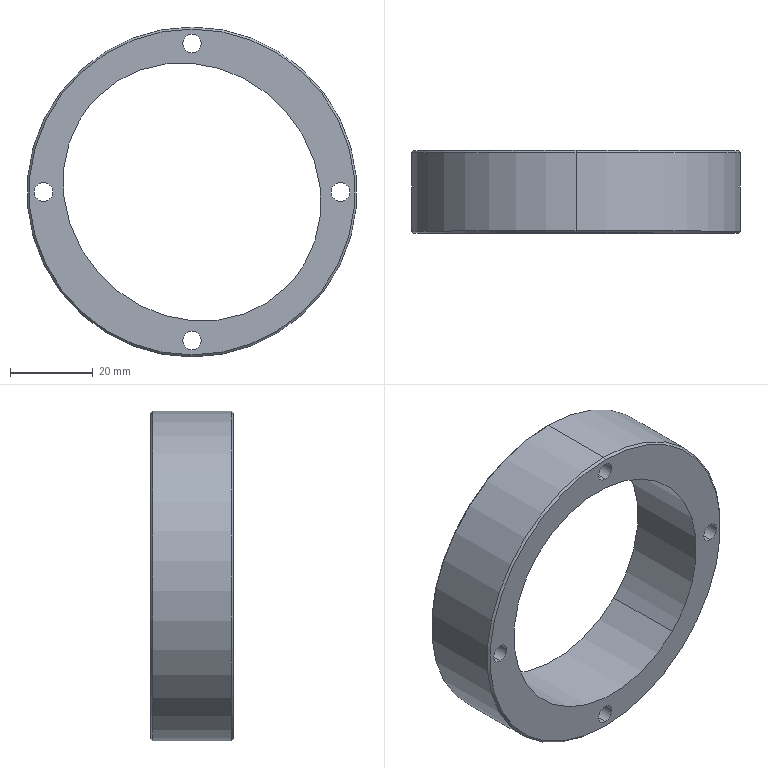Component | SolidWorks | 2-1 | 1 solid | 18 faces | box 80 x 20 x 80 mm | volume 37935 mm3 | cylinder 10 | cone 4 | spline 2 | plane 2 | commonest cylinder face diameters 4.5 x8 80 x2
build123d program:
from build123d import *

# Parameters (mm, degrees)
SKETCH1_R           = 40
BOSS_EXTRUDE1_DEPTH = 20
SKETCH2_R           = 2.25
CUT_EXTRUDE1_DEPTH  = 110
SKETCH3_RX          = 32.5
SKETCH3_RY          = 30
CUT_EXTRUDE2_DEPTH  = 110
CHAMFER1_SIZE       = 0.5


with BuildPart() as part:
    # Sketch1 → Boss-Extrude1 (new body)
    with BuildSketch(Plane(origin=(0, 0, 0), x_dir=(1, 0, 0), z_dir=(0, 1, 0))):
        with Locations(Location((0, 0, 0), (0, 0, 270))):
            Circle(SKETCH1_R)
    extrude(amount=BOSS_EXTRUDE1_DEPTH)

    # Sketch2 → Cut-Extrude1 (cut)
    with BuildSketch(Plane(origin=(0, 20, 0), x_dir=(1, 0, 0), z_dir=(0, 1, 0))):
        with Locations(Location((0, 36, 0), (0, 0, 270))):
            Circle(SKETCH2_R)
        with Locations(Location((36, 0, 0), (0, 0, 270))):
            Circle(SKETCH2_R)
        with Locations(Location((0, -36, 0), (0, 0, 270))):
            Circle(SKETCH2_R)
        with Locations(Location((-36, 0, 0), (0, 0, 270))):
            Circle(SKETCH2_R)
    extrude(amount=-CUT_EXTRUDE1_DEPTH, mode=Mode.SUBTRACT)

    # Sketch3 → Cut-Extrude2 (cut)
    with BuildSketch(Plane(origin=(0, 20, 0), x_dir=(1, 0, 0), z_dir=(0, 1, 0))):
        with Locations(Location((0, 0), (0, 0, 45))):
            Ellipse(SKETCH3_RX, SKETCH3_RY)
    extrude(amount=-CUT_EXTRUDE2_DEPTH, mode=Mode.SUBTRACT)

    # Chamfer1
    chamfer1_edges = [part.edges().sort_by_distance(p)[0] for p in [
        (0, 0, -40),
        (0, 20, -40),
    ]]
    chamfer(chamfer1_edges, length=CHAMFER1_SIZE)


solid = part.part

# Placed as in the assembly
solid = solid.moved(Location((0.004478, 20, 0), (0, 0, 0)))
STEP:
#1=COLOUR_RGB('',0.7922,0.8196,0.9333);
#2=FILL_AREA_STYLE_COLOUR('',#1);
#3=FILL_AREA_STYLE('',(#2));
#4=SURFACE_STYLE_FILL_AREA(#3);
#5=SURFACE_SIDE_STYLE('',(#4));
#6=SURFACE_STYLE_USAGE(.BOTH.,#5);
#7=PRESENTATION_STYLE_ASSIGNMENT((#6));
#8=CARTESIAN_POINT('',(0.,1.575,1.555));
#9=VERTEX_POINT('',#8);
#10=CARTESIAN_POINT('',(0.,1.575,-1.555));
#11=VERTEX_POINT('',#10);
#12=CARTESIAN_POINT('',(0.,1.575,0.));
#13=DIRECTION('',(0.,1.,0.));
#14=DIRECTION('',(0.,0.,1.));
#15=AXIS2_PLACEMENT_3D('',#12,#13,#14);
#16=CIRCLE('',#15,1.555);
#17=EDGE_CURVE('',#9,#11,#16,.T.);
#18=ORIENTED_EDGE('',*,*,#17,.F.);
#19=CARTESIAN_POINT('',(0.,1.555,1.575));
#20=VERTEX_POINT('',#19);
#21=CARTESIAN_POINT('',(0.,1.575,1.555));
#22=DIRECTION('',(0.,-0.7071,0.7071));
#23=VECTOR('',#22,39.37);
#24=LINE('',#21,#23);
#25=EDGE_CURVE('',#9,#20,#24,.T.);
#26=ORIENTED_EDGE('',*,*,#25,.T.);
#27=CARTESIAN_POINT('',(0.,1.555,-1.575));
#28=VERTEX_POINT('',#27);
#29=CARTESIAN_POINT('',(0.,1.555,0.));
#30=DIRECTION('',(0.,-1.,0.));
#31=DIRECTION('',(0.,0.,1.));
#32=AXIS2_PLACEMENT_3D('',#29,#30,#31);
#33=CIRCLE('',#32,1.575);
#34=EDGE_CURVE('',#28,#20,#33,.T.);
#35=ORIENTED_EDGE('',*,*,#34,.F.);
#36=CARTESIAN_POINT('',(0.,1.575,-1.555));
#37=DIRECTION('',(0.,-0.7071,-0.7071));
#38=VECTOR('',#37,39.37);
#39=LINE('',#36,#38);
#40=EDGE_CURVE('',#11,#28,#39,.T.);
#41=ORIENTED_EDGE('',*,*,#40,.F.);
#42=EDGE_LOOP('',(#18,#26,#35,#41));
#43=FACE_OUTER_BOUND('',#42,.T.);
#44=CARTESIAN_POINT('',(0.,1.575,0.));
#45=DIRECTION('',(0.,-1.,0.));
#46=DIRECTION('',(0.,0.,-1.));
#47=AXIS2_PLACEMENT_3D('',#44,#45,#46);
#48=CONICAL_SURFACE('',#47,1.555,0.7854);
#49=ADVANCED_FACE('',(#43),#48,.T.);
#50=CARTESIAN_POINT('',(0.,0.7874,-1.555));
#51=VERTEX_POINT('',#50);
#52=CARTESIAN_POINT('',(0.,0.7874,1.555));
#53=VERTEX_POINT('',#52);
#54=CARTESIAN_POINT('',(0.,0.7874,0.));
#55=DIRECTION('',(0.,-1.,0.));
#56=DIRECTION('',(0.,0.,1.));
#57=AXIS2_PLACEMENT_3D('',#54,#55,#56);
#58=CIRCLE('',#57,1.555);
#59=EDGE_CURVE('',#51,#53,#58,.T.);
#60=ORIENTED_EDGE('',*,*,#59,.F.);
#61=CARTESIAN_POINT('',(0.,0.8071,-1.575));
#62=VERTEX_POINT('',#61);
#63=CARTESIAN_POINT('',(0.,0.8071,-1.575));
#64=DIRECTION('',(0.,0.7071,-0.7071));
#65=VECTOR('',#64,39.37);
#66=LINE('',#63,#65);
#67=EDGE_CURVE('',#51,#62,#66,.T.);
#68=ORIENTED_EDGE('',*,*,#67,.T.);
#69=CARTESIAN_POINT('',(0.,0.8071,1.575));
#70=VERTEX_POINT('',#69);
#71=CARTESIAN_POINT('',(0.,0.8071,0.));
#72=DIRECTION('',(0.,1.,0.));
#73=DIRECTION('',(0.,0.,1.));
#74=AXIS2_PLACEMENT_3D('',#71,#72,#73);
#75=CIRCLE('',#74,1.575);
#76=EDGE_CURVE('',#70,#62,#75,.T.);
#77=ORIENTED_EDGE('',*,*,#76,.F.);
#78=CARTESIAN_POINT('',(0.,0.8071,1.575));
#79=DIRECTION('',(0.,0.7071,0.7071));
#80=VECTOR('',#79,39.37);
#81=LINE('',#78,#80);
#82=EDGE_CURVE('',#53,#70,#81,.T.);
#83=ORIENTED_EDGE('',*,*,#82,.F.);
#84=EDGE_LOOP('',(#60,#68,#77,#83));
#85=FACE_OUTER_BOUND('',#84,.T.);
#86=CARTESIAN_POINT('',(0.,0.8071,0.));
#87=DIRECTION('',(0.,1.,0.));
#88=DIRECTION('',(0.,0.,1.));
#89=AXIS2_PLACEMENT_3D('',#86,#87,#88);
#90=CONICAL_SURFACE('',#89,1.575,0.7854);
#91=ADVANCED_FACE('',(#85),#90,.T.);
#92=CARTESIAN_POINT('',(-0.9048,0.7874,0.9048));
#93=VERTEX_POINT('',#92);
#94=CARTESIAN_POINT('',(0.9048,0.7874,-0.9048));
#95=VERTEX_POINT('',#94);
#96=CARTESIAN_POINT('',(-0.9048,0.7874,0.9048));
#97=CARTESIAN_POINT('',(0.7656,0.7874,2.575));
#98=CARTESIAN_POINT('',(2.575,0.7874,0.7656));
#99=CARTESIAN_POINT('',(0.9048,0.7874,-0.9048));
#100=(BOUNDED_CURVE()B_SPLINE_CURVE(3,(#96,#97,#98,#99),.UNSPECIFIED.,.F.,.F.)B_SPLINE_CURVE_WITH_KNOTS((4,4),(3.142,6.283),.UNSPECIFIED.)CURVE()GEOMETRIC_REPRESENTATION_ITEM()RATIONAL_B_SPLINE_CURVE((1.,0.3333,0.3333,1.))REPRESENTATION_ITEM(''));
#101=EDGE_CURVE('',#93,#95,#100,.T.);
#102=ORIENTED_EDGE('',*,*,#101,.F.);
#103=CARTESIAN_POINT('',(-0.9048,1.575,0.9048));
#104=VERTEX_POINT('',#103);
#105=CARTESIAN_POINT('',(-0.9048,-2.756,0.9048));
#106=DIRECTION('',(0.,1.,0.));
#107=VECTOR('',#106,39.37);
#108=LINE('',#105,#107);
#109=EDGE_CURVE('',#93,#104,#108,.T.);
#110=ORIENTED_EDGE('',*,*,#109,.T.);
#111=CARTESIAN_POINT('',(0.9048,1.575,-0.9048));
#112=VERTEX_POINT('',#111);
#113=CARTESIAN_POINT('',(-0.9048,1.575,0.9048));
#114=CARTESIAN_POINT('',(0.7656,1.575,2.575));
#115=CARTESIAN_POINT('',(2.575,1.575,0.7656));
#116=CARTESIAN_POINT('',(0.9048,1.575,-0.9048));
#117=(BOUNDED_CURVE()B_SPLINE_CURVE(3,(#113,#114,#115,#116),.UNSPECIFIED.,.F.,.F.)B_SPLINE_CURVE_WITH_KNOTS((4,4),(3.142,6.283),.UNSPECIFIED.)CURVE()GEOMETRIC_REPRESENTATION_ITEM()RATIONAL_B_SPLINE_CURVE((1.,0.3333,0.3333,1.))REPRESENTATION_ITEM(''));
#118=EDGE_CURVE('',#104,#112,#117,.T.);
#119=ORIENTED_EDGE('',*,*,#118,.T.);
#120=CARTESIAN_POINT('',(0.9048,-2.756,-0.9048));
#121=DIRECTION('',(0.,1.,0.));
#122=VECTOR('',#121,39.37);
#123=LINE('',#120,#122);
#124=EDGE_CURVE('',#95,#112,#123,.T.);
#125=ORIENTED_EDGE('',*,*,#124,.F.);
#126=EDGE_LOOP('',(#102,#110,#119,#125));
#127=FACE_OUTER_BOUND('',#126,.T.);
#128=CARTESIAN_POINT('',(-0.9048,0.7874,0.9048));
#129=CARTESIAN_POINT('',(-0.9048,1.575,0.9048));
#130=CARTESIAN_POINT('',(0.7656,0.7874,2.575));
#131=CARTESIAN_POINT('',(0.7656,1.575,2.575));
#132=CARTESIAN_POINT('',(2.575,0.7874,0.7656));
#133=CARTESIAN_POINT('',(2.575,1.575,0.7656));
#134=CARTESIAN_POINT('',(0.9048,0.7874,-0.9048));
#135=CARTESIAN_POINT('',(0.9048,1.575,-0.9048));
#136=(BOUNDED_SURFACE()B_SPLINE_SURFACE(3,1,((#128,#129),(#130,#131),(#132,#133),(#134,#135)),.UNSPECIFIED.,.F.,.F.,.F.)B_SPLINE_SURFACE_WITH_KNOTS((4,4),(2,2),(0.,1.),(0.,1.),.UNSPECIFIED.)GEOMETRIC_REPRESENTATION_ITEM()RATIONAL_B_SPLINE_SURFACE(((1.,1.),(0.3333,0.3333),(0.3333,0.3333),(1.,1.)))REPRESENTATION_ITEM('')SURFACE());
#137=ADVANCED_FACE('',(#127),#136,.F.);
#138=CARTESIAN_POINT('',(0.,0.7874,-1.506));
#139=VERTEX_POINT('',#138);
#140=CARTESIAN_POINT('',(0.,0.7874,-1.329));
#141=VERTEX_POINT('',#140);
#142=CARTESIAN_POINT('',(0.,0.7874,-1.417));
#143=DIRECTION('',(0.,1.,0.));
#144=DIRECTION('',(0.,0.,1.));
#145=AXIS2_PLACEMENT_3D('',#142,#143,#144);
#146=CIRCLE('',#145,0.08858);
#147=EDGE_CURVE('',#139,#141,#146,.T.);
#148=ORIENTED_EDGE('',*,*,#147,.F.);
#149=CARTESIAN_POINT('',(0.,1.575,-1.506));
#150=VERTEX_POINT('',#149);
#151=CARTESIAN_POINT('',(0.,-2.756,-1.506));
#152=DIRECTION('',(0.,1.,0.));
#153=VECTOR('',#152,39.37);
#154=LINE('',#151,#153);
#155=EDGE_CURVE('',#139,#150,#154,.T.);
#156=ORIENTED_EDGE('',*,*,#155,.T.);
#157=CARTESIAN_POINT('',(0.,1.575,-1.329));
#158=VERTEX_POINT('',#157);
#159=CARTESIAN_POINT('',(0.,1.575,-1.417));
#160=DIRECTION('',(0.,1.,0.));
#161=DIRECTION('',(0.,0.,1.));
#162=AXIS2_PLACEMENT_3D('',#159,#160,#161);
#163=CIRCLE('',#162,0.08858);
#164=EDGE_CURVE('',#150,#158,#163,.T.);
#165=ORIENTED_EDGE('',*,*,#164,.T.);
#166=CARTESIAN_POINT('',(0.,-2.756,-1.329));
#167=DIRECTION('',(0.,1.,0.));
#168=VECTOR('',#167,39.37);
#169=LINE('',#166,#168);
#170=EDGE_CURVE('',#141,#158,#169,.T.);
#171=ORIENTED_EDGE('',*,*,#170,.F.);
#172=EDGE_LOOP('',(#148,#156,#165,#171));
#173=FACE_OUTER_BOUND('',#172,.T.);
#174=CARTESIAN_POINT('',(0.,-2.756,-1.417));
#175=DIRECTION('',(0.,1.,0.));
#176=DIRECTION('',(0.,0.,1.));
#177=AXIS2_PLACEMENT_3D('',#174,#175,#176);
#178=CYLINDRICAL_SURFACE('',#177,0.08858);
#179=ADVANCED_FACE('',(#173),#178,.F.);
#180=CARTESIAN_POINT('',(1.417,0.7874,-0.08858));
#181=VERTEX_POINT('',#180);
#182=CARTESIAN_POINT('',(1.417,0.7874,0.08858));
#183=VERTEX_POINT('',#182);
#184=CARTESIAN_POINT('',(1.417,0.7874,0.));
#185=DIRECTION('',(0.,1.,0.));
#186=DIRECTION('',(0.,0.,1.));
#187=AXIS2_PLACEMENT_3D('',#184,#185,#186);
#188=CIRCLE('',#187,0.08858);
#189=EDGE_CURVE('',#181,#183,#188,.T.);
#190=ORIENTED_EDGE('',*,*,#189,.F.);
#191=CARTESIAN_POINT('',(1.417,1.575,-0.08858));
#192=VERTEX_POINT('',#191);
#193=CARTESIAN_POINT('',(1.417,-2.756,-0.08858));
#194=DIRECTION('',(0.,1.,0.));
#195=VECTOR('',#194,39.37);
#196=LINE('',#193,#195);
#197=EDGE_CURVE('',#181,#192,#196,.T.);
#198=ORIENTED_EDGE('',*,*,#197,.T.);
#199=CARTESIAN_POINT('',(1.417,1.575,0.08858));
#200=VERTEX_POINT('',#199);
#201=CARTESIAN_POINT('',(1.417,1.575,0.));
#202=DIRECTION('',(0.,1.,0.));
#203=DIRECTION('',(0.,0.,1.));
#204=AXIS2_PLACEMENT_3D('',#201,#202,#203);
#205=CIRCLE('',#204,0.08858);
#206=EDGE_CURVE('',#192,#200,#205,.T.);
#207=ORIENTED_EDGE('',*,*,#206,.T.);
#208=CARTESIAN_POINT('',(1.417,-2.756,0.08858));
#209=DIRECTION('',(0.,1.,0.));
#210=VECTOR('',#209,39.37);
#211=LINE('',#208,#210);
#212=EDGE_CURVE('',#183,#200,#211,.T.);
#213=ORIENTED_EDGE('',*,*,#212,.F.);
#214=EDGE_LOOP('',(#190,#198,#207,#213));
#215=FACE_OUTER_BOUND('',#214,.T.);
#216=CARTESIAN_POINT('',(1.417,-2.756,0.));
#217=DIRECTION('',(0.,1.,0.));
#218=DIRECTION('',(0.,0.,1.));
#219=AXIS2_PLACEMENT_3D('',#216,#217,#218);
#220=CYLINDRICAL_SURFACE('',#219,0.08858);
#221=ADVANCED_FACE('',(#215),#220,.F.);
#222=CARTESIAN_POINT('',(0.,0.7874,1.329));
#223=VERTEX_POINT('',#222);
#224=CARTESIAN_POINT('',(0.,0.7874,1.506));
#225=VERTEX_POINT('',#224);
#226=CARTESIAN_POINT('',(0.,0.7874,1.417));
#227=DIRECTION('',(0.,1.,0.));
#228=DIRECTION('',(0.,0.,1.));
#229=AXIS2_PLACEMENT_3D('',#226,#227,#228);
#230=CIRCLE('',#229,0.08858);
#231=EDGE_CURVE('',#223,#225,#230,.T.);
#232=ORIENTED_EDGE('',*,*,#231,.F.);
#233=CARTESIAN_POINT('',(0.,1.575,1.329));
#234=VERTEX_POINT('',#233);
#235=CARTESIAN_POINT('',(0.,-2.756,1.329));
#236=DIRECTION('',(0.,1.,0.));
#237=VECTOR('',#236,39.37);
#238=LINE('',#235,#237);
#239=EDGE_CURVE('',#223,#234,#238,.T.);
#240=ORIENTED_EDGE('',*,*,#239,.T.);
#241=CARTESIAN_POINT('',(0.,1.575,1.506));
#242=VERTEX_POINT('',#241);
#243=CARTESIAN_POINT('',(0.,1.575,1.417));
#244=DIRECTION('',(0.,1.,0.));
#245=DIRECTION('',(0.,0.,1.));
#246=AXIS2_PLACEMENT_3D('',#243,#244,#245);
#247=CIRCLE('',#246,0.08858);
#248=EDGE_CURVE('',#234,#242,#247,.T.);
#249=ORIENTED_EDGE('',*,*,#248,.T.);
#250=CARTESIAN_POINT('',(0.,-2.756,1.506));
#251=DIRECTION('',(0.,1.,0.));
#252=VECTOR('',#251,39.37);
#253=LINE('',#250,#252);
#254=EDGE_CURVE('',#225,#242,#253,.T.);
#255=ORIENTED_EDGE('',*,*,#254,.F.);
#256=EDGE_LOOP('',(#232,#240,#249,#255));
#257=FACE_OUTER_BOUND('',#256,.T.);
#258=CARTESIAN_POINT('',(0.,-2.756,1.417));
#259=DIRECTION('',(0.,1.,0.));
#260=DIRECTION('',(0.,0.,1.));
#261=AXIS2_PLACEMENT_3D('',#258,#259,#260);
#262=CYLINDRICAL_SURFACE('',#261,0.08858);
#263=ADVANCED_FACE('',(#257),#262,.F.);
#264=CARTESIAN_POINT('',(-1.417,0.7874,-0.08858));
#265=VERTEX_POINT('',#264);
#266=CARTESIAN_POINT('',(-1.417,0.7874,0.08858));
#267=VERTEX_POINT('',#266);
#268=CARTESIAN_POINT('',(-1.417,0.7874,0.));
#269=DIRECTION('',(0.,1.,0.));
#270=DIRECTION('',(0.,0.,1.));
#271=AXIS2_PLACEMENT_3D('',#268,#269,#270);
#272=CIRCLE('',#271,0.08858);
#273=EDGE_CURVE('',#265,#267,#272,.T.);
#274=ORIENTED_EDGE('',*,*,#273,.F.);
#275=CARTESIAN_POINT('',(-1.417,1.575,-0.08858));
#276=VERTEX_POINT('',#275);
#277=CARTESIAN_POINT('',(-1.417,-2.756,-0.08858));
#278=DIRECTION('',(0.,1.,0.));
#279=VECTOR('',#278,39.37);
#280=LINE('',#277,#279);
#281=EDGE_CURVE('',#265,#276,#280,.T.);
#282=ORIENTED_EDGE('',*,*,#281,.T.);
#283=CARTESIAN_POINT('',(-1.417,1.575,0.08858));
#284=VERTEX_POINT('',#283);
#285=CARTESIAN_POINT('',(-1.417,1.575,0.));
#286=DIRECTION('',(0.,1.,0.));
#287=DIRECTION('',(0.,0.,1.));
#288=AXIS2_PLACEMENT_3D('',#285,#286,#287);
#289=CIRCLE('',#288,0.08858);
#290=EDGE_CURVE('',#276,#284,#289,.T.);
#291=ORIENTED_EDGE('',*,*,#290,.T.);
#292=CARTESIAN_POINT('',(-1.417,-2.756,0.08858));
#293=DIRECTION('',(0.,1.,0.));
#294=VECTOR('',#293,39.37);
#295=LINE('',#292,#294);
#296=EDGE_CURVE('',#267,#284,#295,.T.);
#297=ORIENTED_EDGE('',*,*,#296,.F.);
#298=EDGE_LOOP('',(#274,#282,#291,#297));
#299=FACE_OUTER_BOUND('',#298,.T.);
#300=CARTESIAN_POINT('',(-1.417,-2.756,0.));
#301=DIRECTION('',(0.,1.,0.));
#302=DIRECTION('',(0.,0.,1.));
#303=AXIS2_PLACEMENT_3D('',#300,#301,#302);
#304=CYLINDRICAL_SURFACE('',#303,0.08858);
#305=ADVANCED_FACE('',(#299),#304,.F.);
#306=ORIENTED_EDGE('',*,*,#34,.T.);
#307=CARTESIAN_POINT('',(0.,1.575,1.575));
#308=DIRECTION('',(0.,-1.,0.));
#309=VECTOR('',#308,39.37);
#310=LINE('',#307,#309);
#311=EDGE_CURVE('',#20,#70,#310,.T.);
#312=ORIENTED_EDGE('',*,*,#311,.T.);
#313=ORIENTED_EDGE('',*,*,#76,.T.);
#314=CARTESIAN_POINT('',(0.,1.575,-1.575));
#315=DIRECTION('',(0.,-1.,0.));
#316=VECTOR('',#315,39.37);
#317=LINE('',#314,#316);
#318=EDGE_CURVE('',#28,#62,#317,.T.);
#319=ORIENTED_EDGE('',*,*,#318,.F.);
#320=EDGE_LOOP('',(#306,#312,#313,#319));
#321=FACE_OUTER_BOUND('',#320,.T.);
#322=CARTESIAN_POINT('',(0.,1.575,0.));
#323=DIRECTION('',(0.,-1.,0.));
#324=DIRECTION('',(0.,0.,-1.));
#325=AXIS2_PLACEMENT_3D('',#322,#323,#324);
#326=CYLINDRICAL_SURFACE('',#325,1.575);
#327=ADVANCED_FACE('',(#321),#326,.T.);
#328=ORIENTED_EDGE('',*,*,#311,.F.);
#329=CARTESIAN_POINT('',(0.,1.555,0.));
#330=DIRECTION('',(0.,-1.,0.));
#331=DIRECTION('',(0.,0.,1.));
#332=AXIS2_PLACEMENT_3D('',#329,#330,#331);
#333=CIRCLE('',#332,1.575);
#334=EDGE_CURVE('',#20,#28,#333,.T.);
#335=ORIENTED_EDGE('',*,*,#334,.T.);
#336=ORIENTED_EDGE('',*,*,#318,.T.);
#337=CARTESIAN_POINT('',(0.,0.8071,0.));
#338=DIRECTION('',(0.,1.,0.));
#339=DIRECTION('',(0.,0.,1.));
#340=AXIS2_PLACEMENT_3D('',#337,#338,#339);
#341=CIRCLE('',#340,1.575);
#342=EDGE_CURVE('',#62,#70,#341,.T.);
#343=ORIENTED_EDGE('',*,*,#342,.T.);
#344=EDGE_LOOP('',(#328,#335,#336,#343));
#345=FACE_OUTER_BOUND('',#344,.T.);
#346=CARTESIAN_POINT('',(0.,1.575,0.));
#347=DIRECTION('',(0.,-1.,0.));
#348=DIRECTION('',(0.,0.,-1.));
#349=AXIS2_PLACEMENT_3D('',#346,#347,#348);
#350=CYLINDRICAL_SURFACE('',#349,1.575);
#351=ADVANCED_FACE('',(#345),#350,.T.);
#352=CARTESIAN_POINT('',(0.,1.575,0.));
#353=DIRECTION('',(0.,1.,0.));
#354=DIRECTION('',(0.,0.,1.));
#355=AXIS2_PLACEMENT_3D('',#352,#353,#354);
#356=CIRCLE('',#355,1.555);
#357=EDGE_CURVE('',#11,#9,#356,.T.);
#358=ORIENTED_EDGE('',*,*,#357,.T.);
#359=ORIENTED_EDGE('',*,*,#17,.T.);
#360=EDGE_LOOP('',(#358,#359));
#361=FACE_OUTER_BOUND('',#360,.T.);
#362=CARTESIAN_POINT('',(0.9048,1.575,-0.9048));
#363=CARTESIAN_POINT('',(-0.7656,1.575,-2.575));
#364=CARTESIAN_POINT('',(-2.575,1.575,-0.7656));
#365=CARTESIAN_POINT('',(-0.9048,1.575,0.9048));
#366=(BOUNDED_CURVE()B_SPLINE_CURVE(3,(#362,#363,#364,#365),.UNSPECIFIED.,.F.,.T.)B_SPLINE_CURVE_WITH_KNOTS((4,4),(0.,3.142),.UNSPECIFIED.)CURVE()GEOMETRIC_REPRESENTATION_ITEM()RATIONAL_B_SPLINE_CURVE((1.,0.3333,0.3333,1.))REPRESENTATION_ITEM(''));
#367=EDGE_CURVE('',#112,#104,#366,.T.);
#368=ORIENTED_EDGE('',*,*,#367,.F.);
#369=ORIENTED_EDGE('',*,*,#118,.F.);
#370=EDGE_LOOP('',(#368,#369));
#371=FACE_BOUND('',#370,.T.);
#372=CARTESIAN_POINT('',(0.,1.575,-1.417));
#373=DIRECTION('',(0.,1.,0.));
#374=DIRECTION('',(0.,0.,1.));
#375=AXIS2_PLACEMENT_3D('',#372,#373,#374);
#376=CIRCLE('',#375,0.08858);
#377=EDGE_CURVE('',#158,#150,#376,.T.);
#378=ORIENTED_EDGE('',*,*,#377,.F.);
#379=ORIENTED_EDGE('',*,*,#164,.F.);
#380=EDGE_LOOP('',(#378,#379));
#381=FACE_BOUND('',#380,.T.);
#382=CARTESIAN_POINT('',(1.417,1.575,0.));
#383=DIRECTION('',(0.,1.,0.));
#384=DIRECTION('',(0.,0.,1.));
#385=AXIS2_PLACEMENT_3D('',#382,#383,#384);
#386=CIRCLE('',#385,0.08858);
#387=EDGE_CURVE('',#200,#192,#386,.T.);
#388=ORIENTED_EDGE('',*,*,#387,.F.);
#389=ORIENTED_EDGE('',*,*,#206,.F.);
#390=EDGE_LOOP('',(#388,#389));
#391=FACE_BOUND('',#390,.T.);
#392=CARTESIAN_POINT('',(0.,1.575,1.417));
#393=DIRECTION('',(0.,1.,0.));
#394=DIRECTION('',(0.,0.,1.));
#395=AXIS2_PLACEMENT_3D('',#392,#393,#394);
#396=CIRCLE('',#395,0.08858);
#397=EDGE_CURVE('',#242,#234,#396,.T.);
#398=ORIENTED_EDGE('',*,*,#397,.F.);
#399=ORIENTED_EDGE('',*,*,#248,.F.);
#400=EDGE_LOOP('',(#398,#399));
#401=FACE_BOUND('',#400,.T.);
#402=CARTESIAN_POINT('',(-1.417,1.575,0.));
#403=DIRECTION('',(0.,1.,0.));
#404=DIRECTION('',(0.,0.,1.));
#405=AXIS2_PLACEMENT_3D('',#402,#403,#404);
#406=CIRCLE('',#405,0.08858);
#407=EDGE_CURVE('',#284,#276,#406,.T.);
#408=ORIENTED_EDGE('',*,*,#407,.F.);
#409=ORIENTED_EDGE('',*,*,#290,.F.);
#410=EDGE_LOOP('',(#408,#409));
#411=FACE_BOUND('',#410,.T.);
#412=CARTESIAN_POINT('',(0.,1.575,0.));
#413=DIRECTION('',(0.,1.,0.));
#414=DIRECTION('',(0.,0.,1.));
#415=AXIS2_PLACEMENT_3D('',#412,#413,#414);
#416=PLANE('',#415);
#417=ADVANCED_FACE('',(#361,#371,#381,#391,#401,#411),#416,.T.);
#418=CARTESIAN_POINT('',(0.,0.7874,0.));
#419=DIRECTION('',(0.,-1.,0.));
#420=DIRECTION('',(0.,0.,1.));
#421=AXIS2_PLACEMENT_3D('',#418,#419,#420);
#422=CIRCLE('',#421,1.555);
#423=EDGE_CURVE('',#53,#51,#422,.T.);
#424=ORIENTED_EDGE('',*,*,#423,.T.);
#425=ORIENTED_EDGE('',*,*,#59,.T.);
#426=EDGE_LOOP('',(#424,#425));
#427=FACE_OUTER_BOUND('',#426,.T.);
#428=CARTESIAN_POINT('',(0.9048,0.7874,-0.9048));
#429=CARTESIAN_POINT('',(-0.7656,0.7874,-2.575));
#430=CARTESIAN_POINT('',(-2.575,0.7874,-0.7656));
#431=CARTESIAN_POINT('',(-0.9048,0.7874,0.9048));
#432=(BOUNDED_CURVE()B_SPLINE_CURVE(3,(#428,#429,#430,#431),.UNSPECIFIED.,.F.,.F.)B_SPLINE_CURVE_WITH_KNOTS((4,4),(0.,3.142),.UNSPECIFIED.)CURVE()GEOMETRIC_REPRESENTATION_ITEM()RATIONAL_B_SPLINE_CURVE((1.,0.3333,0.3333,1.))REPRESENTATION_ITEM(''));
#433=EDGE_CURVE('',#95,#93,#432,.T.);
#434=ORIENTED_EDGE('',*,*,#433,.T.);
#435=ORIENTED_EDGE('',*,*,#101,.T.);
#436=EDGE_LOOP('',(#434,#435));
#437=FACE_BOUND('',#436,.T.);
#438=CARTESIAN_POINT('',(0.,0.7874,-1.417));
#439=DIRECTION('',(0.,1.,0.));
#440=DIRECTION('',(0.,0.,1.));
#441=AXIS2_PLACEMENT_3D('',#438,#439,#440);
#442=CIRCLE('',#441,0.08858);
#443=EDGE_CURVE('',#141,#139,#442,.T.);
#444=ORIENTED_EDGE('',*,*,#443,.T.);
#445=ORIENTED_EDGE('',*,*,#147,.T.);
#446=EDGE_LOOP('',(#444,#445));
#447=FACE_BOUND('',#446,.T.);
#448=CARTESIAN_POINT('',(1.417,0.7874,0.));
#449=DIRECTION('',(0.,1.,0.));
#450=DIRECTION('',(0.,0.,1.));
#451=AXIS2_PLACEMENT_3D('',#448,#449,#450);
#452=CIRCLE('',#451,0.08858);
#453=EDGE_CURVE('',#183,#181,#452,.T.);
#454=ORIENTED_EDGE('',*,*,#453,.T.);
#455=ORIENTED_EDGE('',*,*,#189,.T.);
#456=EDGE_LOOP('',(#454,#455));
#457=FACE_BOUND('',#456,.T.);
#458=CARTESIAN_POINT('',(0.,0.7874,1.417));
#459=DIRECTION('',(0.,1.,0.));
#460=DIRECTION('',(0.,0.,1.));
#461=AXIS2_PLACEMENT_3D('',#458,#459,#460);
#462=CIRCLE('',#461,0.08858);
#463=EDGE_CURVE('',#225,#223,#462,.T.);
#464=ORIENTED_EDGE('',*,*,#463,.T.);
#465=ORIENTED_EDGE('',*,*,#231,.T.);
#466=EDGE_LOOP('',(#464,#465));
#467=FACE_BOUND('',#466,.T.);
#468=CARTESIAN_POINT('',(-1.417,0.7874,0.));
#469=DIRECTION('',(0.,1.,0.));
#470=DIRECTION('',(0.,0.,1.));
#471=AXIS2_PLACEMENT_3D('',#468,#469,#470);
#472=CIRCLE('',#471,0.08858);
#473=EDGE_CURVE('',#267,#265,#472,.T.);
#474=ORIENTED_EDGE('',*,*,#473,.T.);
#475=ORIENTED_EDGE('',*,*,#273,.T.);
#476=EDGE_LOOP('',(#474,#475));
#477=FACE_BOUND('',#476,.T.);
#478=CARTESIAN_POINT('',(0.,0.7874,0.));
#479=DIRECTION('',(0.,1.,0.));
#480=DIRECTION('',(0.,0.,1.));
#481=AXIS2_PLACEMENT_3D('',#478,#479,#480);
#482=PLANE('',#481);
#483=ADVANCED_FACE('',(#427,#437,#447,#457,#467,#477),#482,.F.);
#484=ORIENTED_EDGE('',*,*,#281,.F.);
#485=ORIENTED_EDGE('',*,*,#473,.F.);
#486=ORIENTED_EDGE('',*,*,#296,.T.);
#487=ORIENTED_EDGE('',*,*,#407,.T.);
#488=EDGE_LOOP('',(#484,#485,#486,#487));
#489=FACE_OUTER_BOUND('',#488,.T.);
#490=CARTESIAN_POINT('',(-1.417,-2.756,0.));
#491=DIRECTION('',(0.,1.,0.));
#492=DIRECTION('',(0.,0.,1.));
#493=AXIS2_PLACEMENT_3D('',#490,#491,#492);
#494=CYLINDRICAL_SURFACE('',#493,0.08858);
#495=ADVANCED_FACE('',(#489),#494,.F.);
#496=ORIENTED_EDGE('',*,*,#239,.F.);
#497=ORIENTED_EDGE('',*,*,#463,.F.);
#498=ORIENTED_EDGE('',*,*,#254,.T.);
#499=ORIENTED_EDGE('',*,*,#397,.T.);
#500=EDGE_LOOP('',(#496,#497,#498,#499));
#501=FACE_OUTER_BOUND('',#500,.T.);
#502=CARTESIAN_POINT('',(0.,-2.756,1.417));
#503=DIRECTION('',(0.,1.,0.));
#504=DIRECTION('',(0.,0.,1.));
#505=AXIS2_PLACEMENT_3D('',#502,#503,#504);
#506=CYLINDRICAL_SURFACE('',#505,0.08858);
#507=ADVANCED_FACE('',(#501),#506,.F.);
#508=ORIENTED_EDGE('',*,*,#197,.F.);
#509=ORIENTED_EDGE('',*,*,#453,.F.);
#510=ORIENTED_EDGE('',*,*,#212,.T.);
#511=ORIENTED_EDGE('',*,*,#387,.T.);
#512=EDGE_LOOP('',(#508,#509,#510,#511));
#513=FACE_OUTER_BOUND('',#512,.T.);
#514=CARTESIAN_POINT('',(1.417,-2.756,0.));
#515=DIRECTION('',(0.,1.,0.));
#516=DIRECTION('',(0.,0.,1.));
#517=AXIS2_PLACEMENT_3D('',#514,#515,#516);
#518=CYLINDRICAL_SURFACE('',#517,0.08858);
#519=ADVANCED_FACE('',(#513),#518,.F.);
#520=ORIENTED_EDGE('',*,*,#155,.F.);
#521=ORIENTED_EDGE('',*,*,#443,.F.);
#522=ORIENTED_EDGE('',*,*,#170,.T.);
#523=ORIENTED_EDGE('',*,*,#377,.T.);
#524=EDGE_LOOP('',(#520,#521,#522,#523));
#525=FACE_OUTER_BOUND('',#524,.T.);
#526=CARTESIAN_POINT('',(0.,-2.756,-1.417));
#527=DIRECTION('',(0.,1.,0.));
#528=DIRECTION('',(0.,0.,1.));
#529=AXIS2_PLACEMENT_3D('',#526,#527,#528);
#530=CYLINDRICAL_SURFACE('',#529,0.08858);
#531=ADVANCED_FACE('',(#525),#530,.F.);
#532=ORIENTED_EDGE('',*,*,#109,.F.);
#533=ORIENTED_EDGE('',*,*,#433,.F.);
#534=ORIENTED_EDGE('',*,*,#124,.T.);
#535=ORIENTED_EDGE('',*,*,#367,.T.);
#536=EDGE_LOOP('',(#532,#533,#534,#535));
#537=FACE_OUTER_BOUND('',#536,.T.);
#538=CARTESIAN_POINT('',(0.9048,0.7874,-0.9048));
#539=CARTESIAN_POINT('',(0.9048,1.575,-0.9048));
#540=CARTESIAN_POINT('',(-0.7656,0.7874,-2.575));
#541=CARTESIAN_POINT('',(-0.7656,1.575,-2.575));
#542=CARTESIAN_POINT('',(-2.575,0.7874,-0.7656));
#543=CARTESIAN_POINT('',(-2.575,1.575,-0.7656));
#544=CARTESIAN_POINT('',(-0.9048,0.7874,0.9048));
#545=CARTESIAN_POINT('',(-0.9048,1.575,0.9048));
#546=(BOUNDED_SURFACE()B_SPLINE_SURFACE(3,1,((#538,#539),(#540,#541),(#542,#543),(#544,#545)),.UNSPECIFIED.,.F.,.F.,.F.)B_SPLINE_SURFACE_WITH_KNOTS((4,4),(2,2),(0.,1.),(0.,1.),.UNSPECIFIED.)GEOMETRIC_REPRESENTATION_ITEM()RATIONAL_B_SPLINE_SURFACE(((1.,1.),(0.3333,0.3333),(0.3333,0.3333),(1.,1.)))REPRESENTATION_ITEM('')SURFACE());
#547=ADVANCED_FACE('',(#537),#546,.F.);
#548=ORIENTED_EDGE('',*,*,#67,.F.);
#549=ORIENTED_EDGE('',*,*,#423,.F.);
#550=ORIENTED_EDGE('',*,*,#82,.T.);
#551=ORIENTED_EDGE('',*,*,#342,.F.);
#552=EDGE_LOOP('',(#548,#549,#550,#551));
#553=FACE_OUTER_BOUND('',#552,.T.);
#554=CARTESIAN_POINT('',(0.,0.8071,0.));
#555=DIRECTION('',(0.,1.,0.));
#556=DIRECTION('',(0.,0.,1.));
#557=AXIS2_PLACEMENT_3D('',#554,#555,#556);
#558=CONICAL_SURFACE('',#557,1.575,0.7854);
#559=ADVANCED_FACE('',(#553),#558,.T.);
#560=ORIENTED_EDGE('',*,*,#25,.F.);
#561=ORIENTED_EDGE('',*,*,#357,.F.);
#562=ORIENTED_EDGE('',*,*,#40,.T.);
#563=ORIENTED_EDGE('',*,*,#334,.F.);
#564=EDGE_LOOP('',(#560,#561,#562,#563));
#565=FACE_OUTER_BOUND('',#564,.T.);
#566=CARTESIAN_POINT('',(0.,1.575,0.));
#567=DIRECTION('',(0.,-1.,0.));
#568=DIRECTION('',(0.,0.,-1.));
#569=AXIS2_PLACEMENT_3D('',#566,#567,#568);
#570=CONICAL_SURFACE('',#569,1.555,0.7854);
#571=ADVANCED_FACE('',(#565),#570,.T.);
#572=CLOSED_SHELL('',(#49,#91,#137,#179,#221,#263,#305,#327,#351,#417,#483,#495,#507,#519,#531,#547,#559,#571));
#573=MANIFOLD_SOLID_BREP('',#572);
#574=STYLED_ITEM('',(#7),#573);
#575=(LENGTH_UNIT()NAMED_UNIT(*)SI_UNIT($,.METRE.));
#576=LENGTH_MEASURE_WITH_UNIT(LENGTH_MEASURE(0.0254),#575);
#577=DIMENSIONAL_EXPONENTS(1.,0.,0.,0.,0.,0.,0.);
#578=(CONVERSION_BASED_UNIT('',#576)LENGTH_UNIT()NAMED_UNIT(#577));
#579=UNCERTAINTY_MEASURE_WITH_UNIT(LENGTH_MEASURE(0.00001),#578,'','');
#580=(NAMED_UNIT(*)PLANE_ANGLE_UNIT()SI_UNIT($,.RADIAN.));
#581=(NAMED_UNIT(*)SI_UNIT($,.STERADIAN.)SOLID_ANGLE_UNIT());
#582=(GEOMETRIC_REPRESENTATION_CONTEXT(3)GLOBAL_UNCERTAINTY_ASSIGNED_CONTEXT((#579))GLOBAL_UNIT_ASSIGNED_CONTEXT((#578,#580,#581))REPRESENTATION_CONTEXT('',''));
#583=MECHANICAL_DESIGN_GEOMETRIC_PRESENTATION_REPRESENTATION('',(#574),#582);
#584=CARTESIAN_POINT('',(0.,0.,0.));
#585=DIRECTION('',(0.,0.,1.));
#586=DIRECTION('',(1.,0.,0.));
#587=AXIS2_PLACEMENT_3D('',#584,#585,#586);
#588=(LENGTH_UNIT()NAMED_UNIT(*)SI_UNIT($,.METRE.));
#589=LENGTH_MEASURE_WITH_UNIT(LENGTH_MEASURE(0.0254),#588);
#590=DIMENSIONAL_EXPONENTS(1.,0.,0.,0.,0.,0.,0.);
#591=(CONVERSION_BASED_UNIT('',#589)LENGTH_UNIT()NAMED_UNIT(#590));
#592=UNCERTAINTY_MEASURE_WITH_UNIT(LENGTH_MEASURE(0.00001),#591,'','');
#593=(NAMED_UNIT(*)PLANE_ANGLE_UNIT()SI_UNIT($,.RADIAN.));
#594=(NAMED_UNIT(*)SI_UNIT($,.STERADIAN.)SOLID_ANGLE_UNIT());
#595=(GEOMETRIC_REPRESENTATION_CONTEXT(3)GLOBAL_UNCERTAINTY_ASSIGNED_CONTEXT((#592))GLOBAL_UNIT_ASSIGNED_CONTEXT((#591,#593,#594))REPRESENTATION_CONTEXT('',''));
#596=ADVANCED_BREP_SHAPE_REPRESENTATION('',(#573,#587),#595);
#597=PRESENTATION_LAYER_ASSIGNMENT('','',(#574));